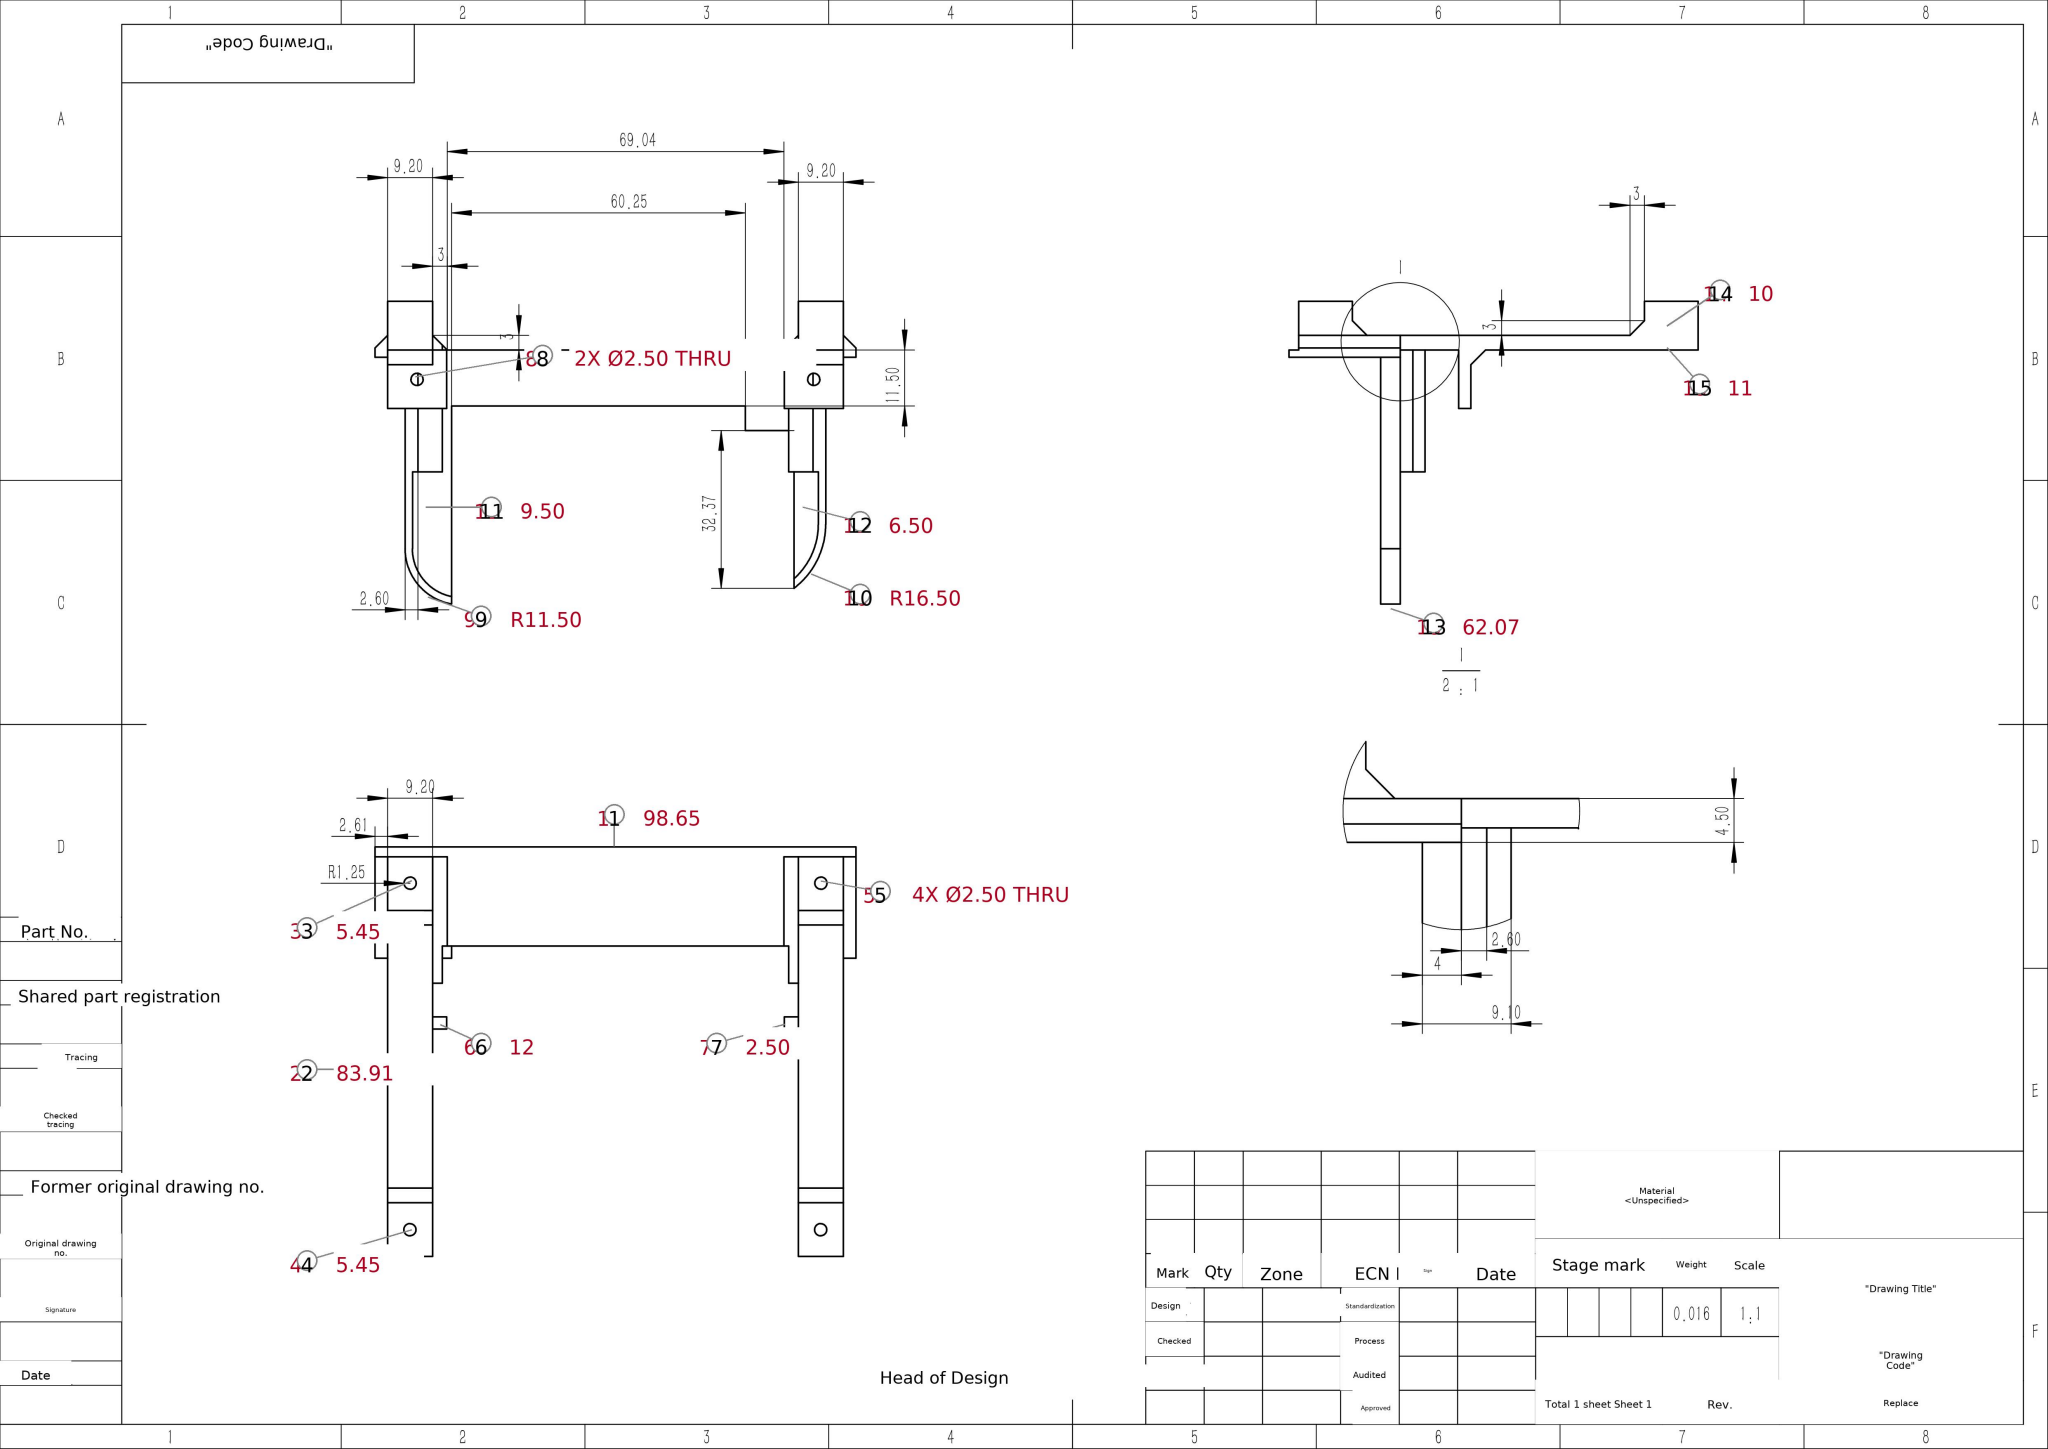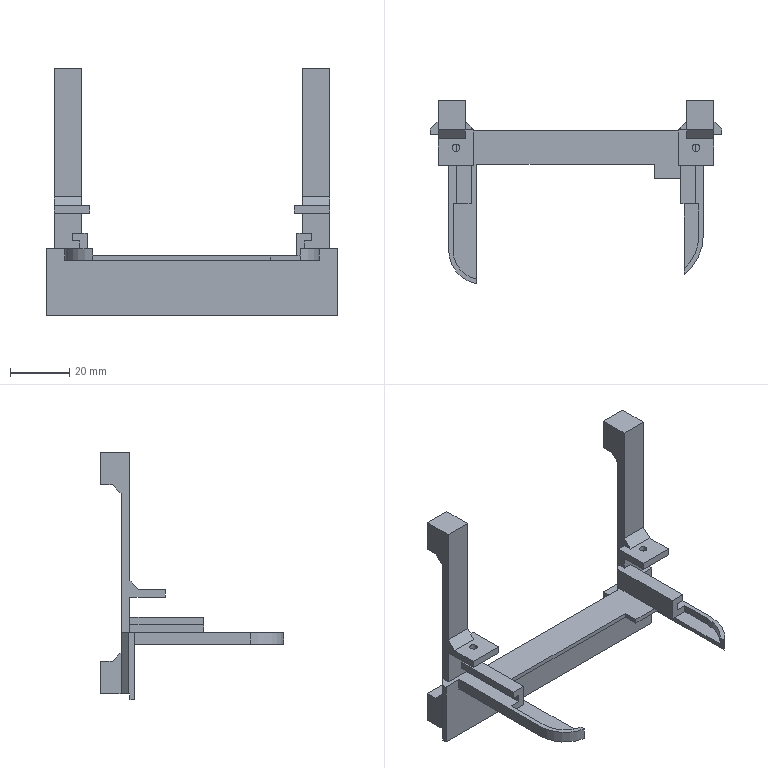Part | SolidWorks | mm | material <Unspecified> | 1 solid | 98 faces | box 98.65 x 62.07 x 83.91 mm | volume 16007 mm3 | plane 82 | cylinder 16 | commonest cylinder face diameters 2.5 x12 23 x1 20 x1 33 x1 30 x1